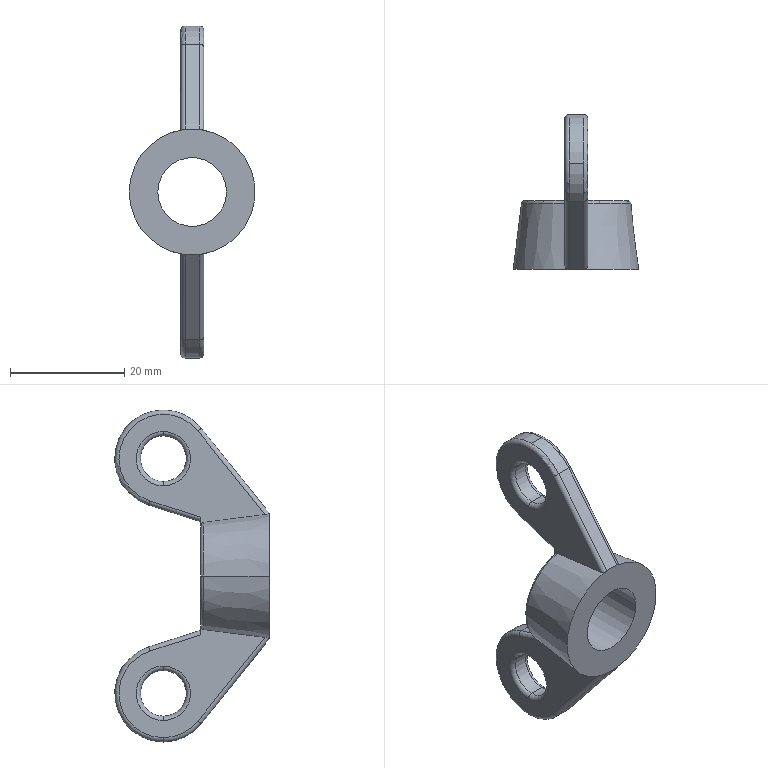Component | SolidWorks | GB_T62.1-2004WingNutRoundWingM12_1.75-1 | 1 solid | 47 faces | volume 4784 mm3 | torus 17 | cylinder 17 | plane 10 | cone 3 | commonest cylinder face diameters 1.5 x8 8 x4 17 x3 12 x2